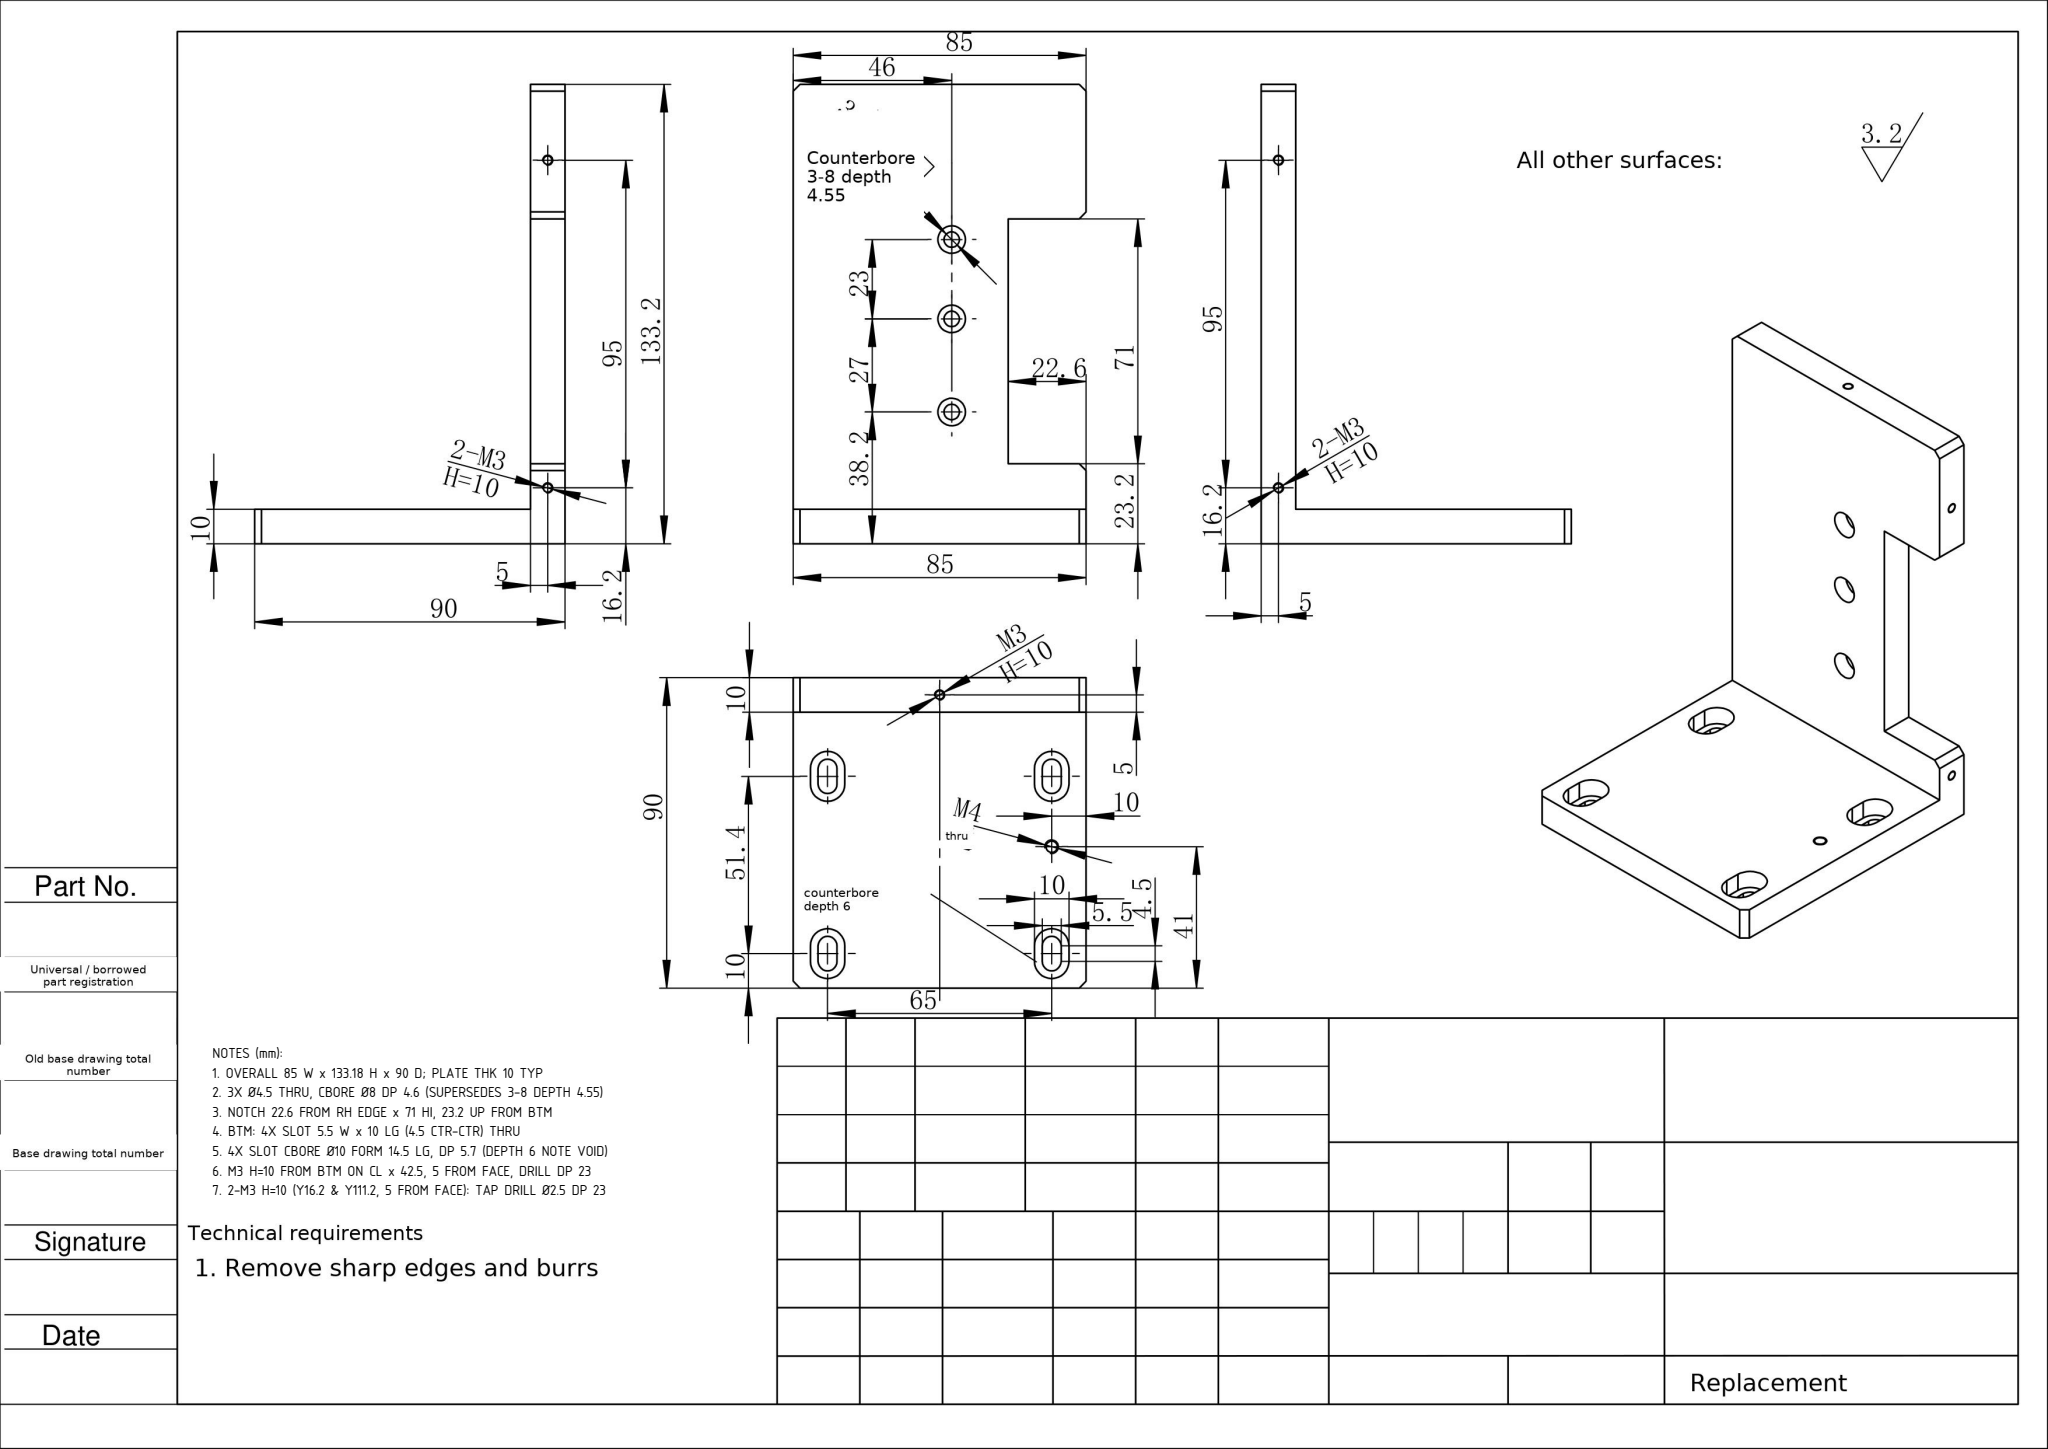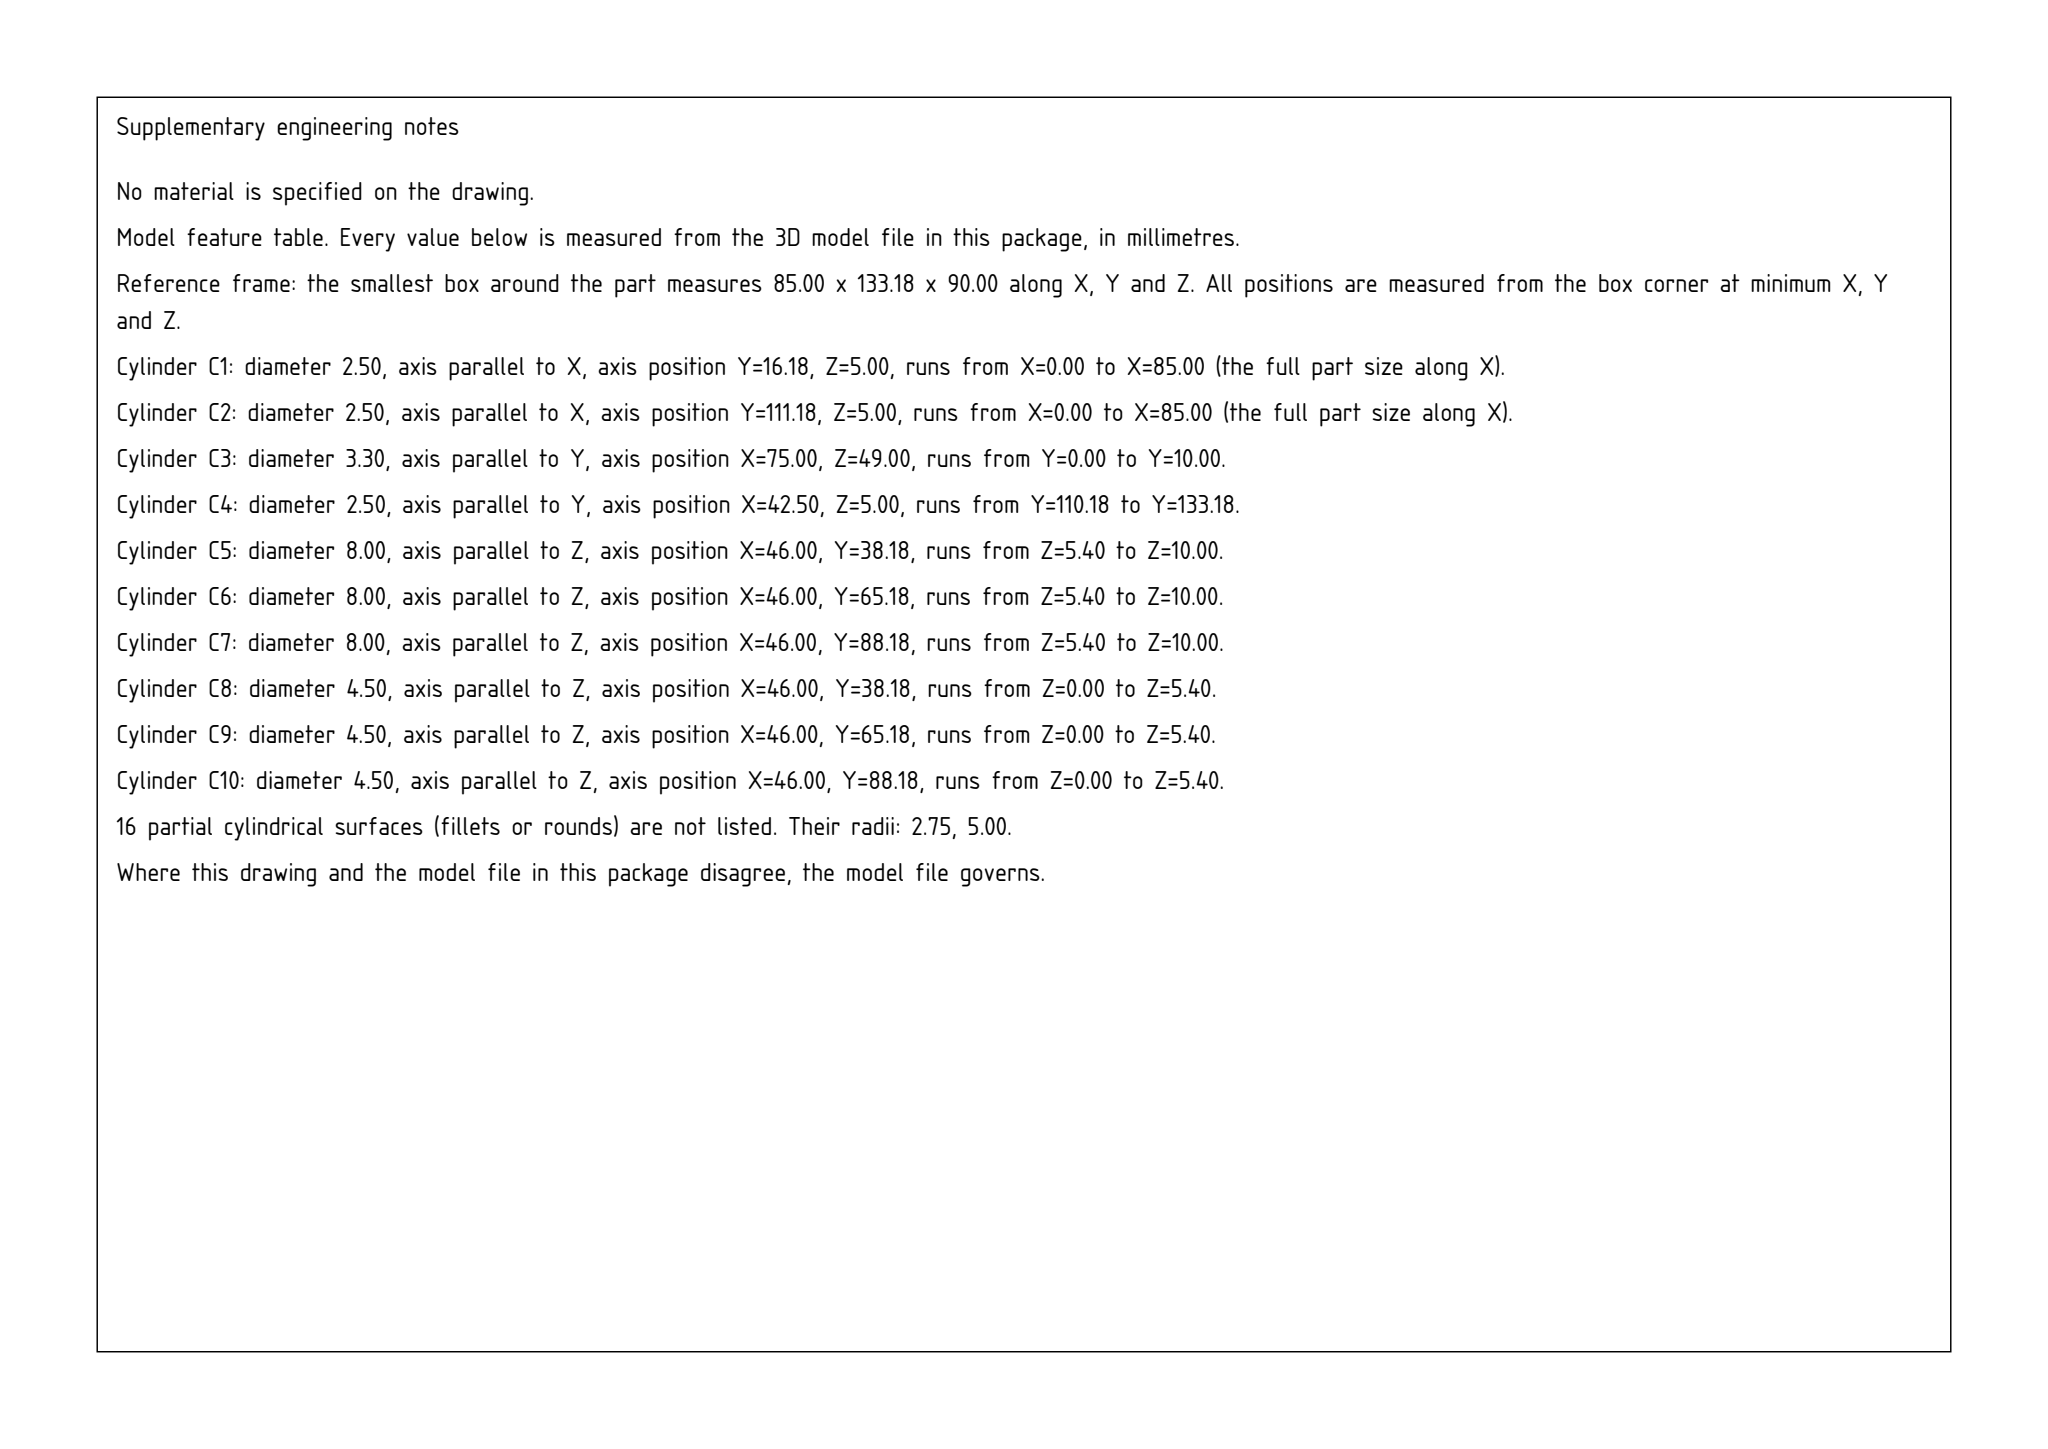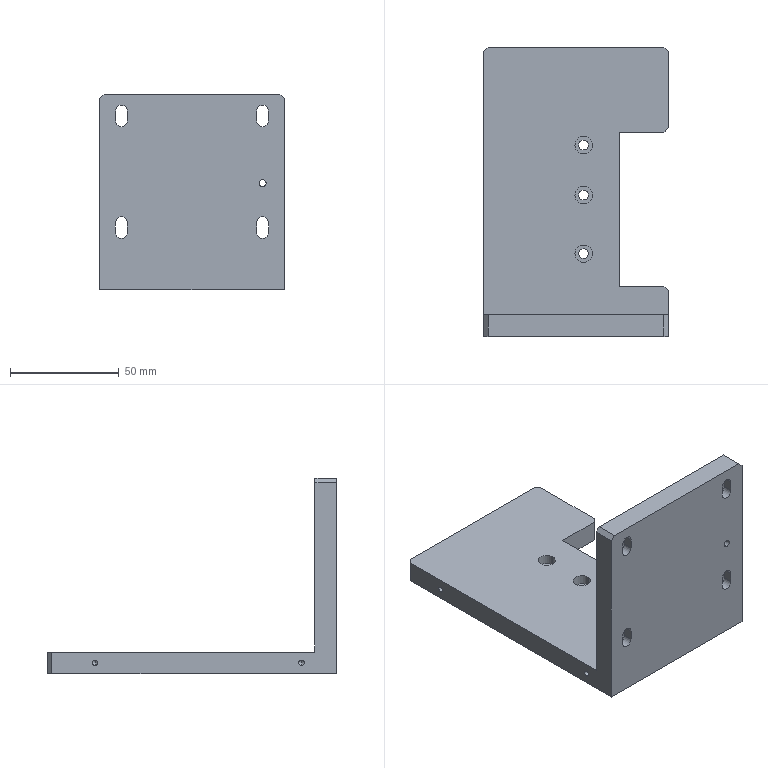Part | SolidWorks | mm | 1 solid | 99 faces | box 85 x 133.18 x 90 mm | volume 159764 mm3 | cylinder 48 | plane 41 | cone 10 | commonest cylinder face diameters 10 x12 5.5 x12 2.5 x10 8 x6 4.5 x6 3.3 x2
Drawing notes:
OVERALL 85 W x 133.18 H x 90 D; PLATE THK 10 TYP | from the solid: bbox 85 x 133.179 x 90; z planes 0/10 (vert plate), y planes 0/10 (base plate)
3X Ø4.5 THRU, CBORE Ø8 DP 4.6 (SUPERSEDES 3-8 DEPTH 4.55) | from the solid: Ø4.5 z-axis len 5.4 + Ø8 z-axis len 4.6 at x=46, y=38.18/65.18/88.18; 5.4+4.6=10 wall
NOTCH 22.6 FROM RH EDGE x 71 HI, 23.2 UP FROM BTM | from the solid: x plane 62.38 (85-62.38=22.62); y planes 23.18 & 94.18, diff = 71
BTM: 4X SLOT 5.5 W x 10 LG (4.5 CTR-CTR) THRU | from the solid: Ø5.5 y-axis at x=10 & 75, z 26.35/30.85 & 77.75/82.25 (4.5 apart), len 4.3
4X SLOT CBORE Ø10 FORM 14.5 LG, DP 5.7 (DEPTH 6 NOTE VOID) | from the solid: Ø10 y-axis cyls on same centres as Ø5.5 slots, len 5.7; 5.7+4.3=10 plate thk
M3 H=10 FROM BTM ON CL x 42.5, 5 FROM FACE, DRILL DP 23 | from the solid: Ø2.5 y-axis cyl at [42.5, null, 5.0], len 23, count 2
2-M3 H=10 (Y16.2 & Y111.2, 5 FROM FACE): TAP DRILL Ø2.5 DP 23 | from the solid: cylinders [2.5,"x",[null,16.18,5.0],23.0] and [2.5,"x",[null,111.18,5.0],23.0]